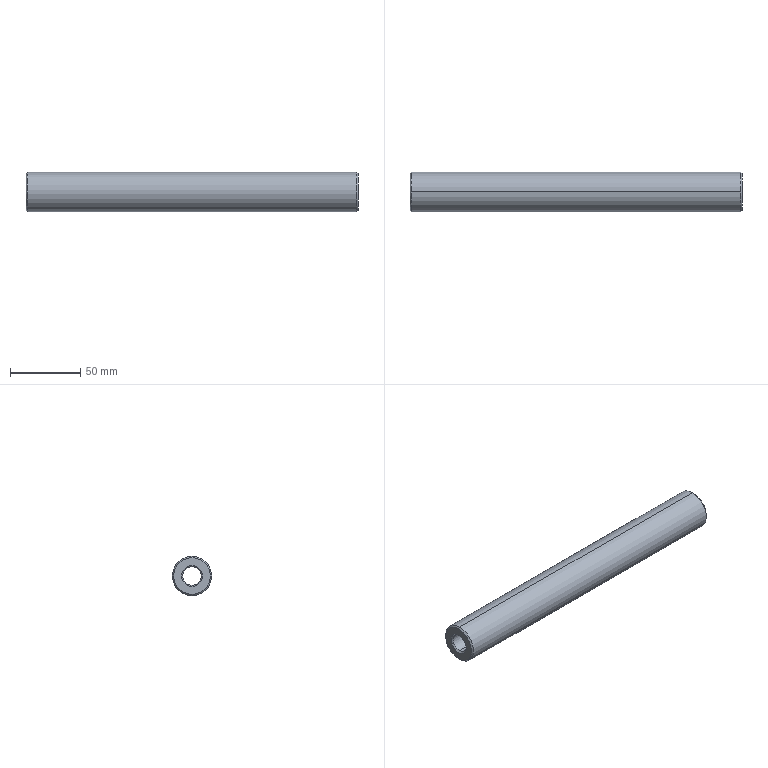Component | SolidWorks | LocatingGuideBushing156-2 | 1 solid | 14 faces | box 236 x 28 x 28 mm | volume 113864 mm3 | cone 8 | cylinder 4 | plane 2 | commonest cylinder face diameters 13 x2 28 x2
build123d program:
from build123d import *

# Parameters (mm, degrees)
SKETCH1_R           = 14
SKETCH1_R_2         = 6.5
BOSS_EXTRUDE1_DEPTH = 236
CHAMFER1_SIZE       = 1


with BuildPart() as part:
    # Sketch1 → Boss-Extrude1 (new body)
    with BuildSketch(Plane.XY):
        Circle(SKETCH1_R)
        Circle(SKETCH1_R_2, mode=Mode.SUBTRACT)
    extrude(amount=BOSS_EXTRUDE1_DEPTH)

    # Chamfer1
    chamfer1_edges = [part.edges().sort_by_distance(p)[0] for p in [
        (-14, 0, 0),
        (-14, 0, 236),
        (-6.5, 0, 0),
        (-6.5, 0, 236),
    ]]
    chamfer(chamfer1_edges, length=CHAMFER1_SIZE)


solid = part.part

# Placed as in the assembly
solid = solid.moved(Location((-455.809, -229.181, 0), (0, 90, 0)))
STEP:
#1=COLOUR_RGB('',0.7922,0.8196,0.9333);
#2=FILL_AREA_STYLE_COLOUR('',#1);
#3=FILL_AREA_STYLE('',(#2));
#4=SURFACE_STYLE_FILL_AREA(#3);
#5=SURFACE_SIDE_STYLE('',(#4));
#6=SURFACE_STYLE_USAGE(.BOTH.,#5);
#7=PRESENTATION_STYLE_ASSIGNMENT((#6));
#8=CARTESIAN_POINT('',(-8.654,-9.023,-0.5118));
#9=VERTEX_POINT('',#8);
#10=CARTESIAN_POINT('',(-8.654,-9.023,0.5118));
#11=VERTEX_POINT('',#10);
#12=CARTESIAN_POINT('',(-8.654,-9.023,-0.));
#13=DIRECTION('',(1.,-0.,0.));
#14=DIRECTION('',(0.,0.,-1.));
#15=AXIS2_PLACEMENT_3D('',#12,#13,#14);
#16=CIRCLE('',#15,0.5118);
#17=EDGE_CURVE('',#9,#11,#16,.T.);
#18=ORIENTED_EDGE('',*,*,#17,.F.);
#19=CARTESIAN_POINT('',(-8.693,-9.023,-0.5512));
#20=VERTEX_POINT('',#19);
#21=CARTESIAN_POINT('',(-8.654,-9.023,-0.5118));
#22=DIRECTION('',(-0.7071,0.,-0.7071));
#23=VECTOR('',#22,39.37);
#24=LINE('',#21,#23);
#25=EDGE_CURVE('',#9,#20,#24,.T.);
#26=ORIENTED_EDGE('',*,*,#25,.T.);
#27=CARTESIAN_POINT('',(-8.693,-9.023,0.5512));
#28=VERTEX_POINT('',#27);
#29=CARTESIAN_POINT('',(-8.693,-9.023,-0.));
#30=DIRECTION('',(-1.,0.,-0.));
#31=DIRECTION('',(0.,0.,-1.));
#32=AXIS2_PLACEMENT_3D('',#29,#30,#31);
#33=CIRCLE('',#32,0.5512);
#34=EDGE_CURVE('',#28,#20,#33,.T.);
#35=ORIENTED_EDGE('',*,*,#34,.F.);
#36=CARTESIAN_POINT('',(-8.654,-9.023,0.5118));
#37=DIRECTION('',(-0.7071,-0.,0.7071));
#38=VECTOR('',#37,39.37);
#39=LINE('',#36,#38);
#40=EDGE_CURVE('',#11,#28,#39,.T.);
#41=ORIENTED_EDGE('',*,*,#40,.F.);
#42=EDGE_LOOP('',(#18,#26,#35,#41));
#43=FACE_OUTER_BOUND('',#42,.T.);
#44=CARTESIAN_POINT('',(-8.654,-9.023,-0.));
#45=DIRECTION('',(-1.,0.,-0.));
#46=DIRECTION('',(0.,0.,1.));
#47=AXIS2_PLACEMENT_3D('',#44,#45,#46);
#48=CONICAL_SURFACE('',#47,0.5118,0.7854);
#49=ADVANCED_FACE('',(#43),#48,.T.);
#50=CARTESIAN_POINT('',(-8.693,-9.023,0.2559));
#51=VERTEX_POINT('',#50);
#52=CARTESIAN_POINT('',(-8.693,-9.023,-0.2559));
#53=VERTEX_POINT('',#52);
#54=CARTESIAN_POINT('',(-8.693,-9.023,-0.));
#55=DIRECTION('',(1.,-0.,0.));
#56=DIRECTION('',(0.,0.,-1.));
#57=AXIS2_PLACEMENT_3D('',#54,#55,#56);
#58=CIRCLE('',#57,0.2559);
#59=EDGE_CURVE('',#51,#53,#58,.T.);
#60=ORIENTED_EDGE('',*,*,#59,.F.);
#61=CARTESIAN_POINT('',(-8.654,-9.023,0.2953));
#62=VERTEX_POINT('',#61);
#63=CARTESIAN_POINT('',(-8.693,-9.023,0.2559));
#64=DIRECTION('',(0.7071,-0.,0.7071));
#65=VECTOR('',#64,39.37);
#66=LINE('',#63,#65);
#67=EDGE_CURVE('',#51,#62,#66,.T.);
#68=ORIENTED_EDGE('',*,*,#67,.T.);
#69=CARTESIAN_POINT('',(-8.654,-9.023,-0.2953));
#70=VERTEX_POINT('',#69);
#71=CARTESIAN_POINT('',(-8.654,-9.023,-0.));
#72=DIRECTION('',(-1.,0.,-0.));
#73=DIRECTION('',(0.,0.,-1.));
#74=AXIS2_PLACEMENT_3D('',#71,#72,#73);
#75=CIRCLE('',#74,0.2953);
#76=EDGE_CURVE('',#70,#62,#75,.T.);
#77=ORIENTED_EDGE('',*,*,#76,.F.);
#78=CARTESIAN_POINT('',(-8.693,-9.023,-0.2559));
#79=DIRECTION('',(0.7071,0.,-0.7071));
#80=VECTOR('',#79,39.37);
#81=LINE('',#78,#80);
#82=EDGE_CURVE('',#53,#70,#81,.T.);
#83=ORIENTED_EDGE('',*,*,#82,.F.);
#84=EDGE_LOOP('',(#60,#68,#77,#83));
#85=FACE_OUTER_BOUND('',#84,.T.);
#86=CARTESIAN_POINT('',(-8.693,-9.023,-0.));
#87=DIRECTION('',(1.,-0.,0.));
#88=DIRECTION('',(0.,0.,-1.));
#89=AXIS2_PLACEMENT_3D('',#86,#87,#88);
#90=CONICAL_SURFACE('',#89,0.2559,0.7854);
#91=ADVANCED_FACE('',(#85),#90,.F.);
#92=CARTESIAN_POINT('',(-17.945,-9.023,0.5118));
#93=VERTEX_POINT('',#92);
#94=CARTESIAN_POINT('',(-17.945,-9.023,-0.5118));
#95=VERTEX_POINT('',#94);
#96=CARTESIAN_POINT('',(-17.945,-9.023,-0.));
#97=DIRECTION('',(-1.,0.,-0.));
#98=DIRECTION('',(0.,0.,-1.));
#99=AXIS2_PLACEMENT_3D('',#96,#97,#98);
#100=CIRCLE('',#99,0.5118);
#101=EDGE_CURVE('',#93,#95,#100,.T.);
#102=ORIENTED_EDGE('',*,*,#101,.F.);
#103=CARTESIAN_POINT('',(-17.906,-9.023,0.5512));
#104=VERTEX_POINT('',#103);
#105=CARTESIAN_POINT('',(-17.906,-9.023,0.5512));
#106=DIRECTION('',(0.7071,-0.,0.7071));
#107=VECTOR('',#106,39.37);
#108=LINE('',#105,#107);
#109=EDGE_CURVE('',#93,#104,#108,.T.);
#110=ORIENTED_EDGE('',*,*,#109,.T.);
#111=CARTESIAN_POINT('',(-17.906,-9.023,-0.5512));
#112=VERTEX_POINT('',#111);
#113=CARTESIAN_POINT('',(-17.906,-9.023,-0.));
#114=DIRECTION('',(1.,-0.,0.));
#115=DIRECTION('',(0.,0.,-1.));
#116=AXIS2_PLACEMENT_3D('',#113,#114,#115);
#117=CIRCLE('',#116,0.5512);
#118=EDGE_CURVE('',#112,#104,#117,.T.);
#119=ORIENTED_EDGE('',*,*,#118,.F.);
#120=CARTESIAN_POINT('',(-17.906,-9.023,-0.5512));
#121=DIRECTION('',(0.7071,0.,-0.7071));
#122=VECTOR('',#121,39.37);
#123=LINE('',#120,#122);
#124=EDGE_CURVE('',#95,#112,#123,.T.);
#125=ORIENTED_EDGE('',*,*,#124,.F.);
#126=EDGE_LOOP('',(#102,#110,#119,#125));
#127=FACE_OUTER_BOUND('',#126,.T.);
#128=CARTESIAN_POINT('',(-17.906,-9.023,-0.));
#129=DIRECTION('',(1.,-0.,0.));
#130=DIRECTION('',(0.,0.,-1.));
#131=AXIS2_PLACEMENT_3D('',#128,#129,#130);
#132=CONICAL_SURFACE('',#131,0.5512,0.7854);
#133=ADVANCED_FACE('',(#127),#132,.T.);
#134=CARTESIAN_POINT('',(-17.906,-9.023,-0.2559));
#135=VERTEX_POINT('',#134);
#136=CARTESIAN_POINT('',(-17.906,-9.023,0.2559));
#137=VERTEX_POINT('',#136);
#138=CARTESIAN_POINT('',(-17.906,-9.023,-0.));
#139=DIRECTION('',(-1.,0.,-0.));
#140=DIRECTION('',(0.,-0.,-1.));
#141=AXIS2_PLACEMENT_3D('',#138,#139,#140);
#142=CIRCLE('',#141,0.2559);
#143=EDGE_CURVE('',#135,#137,#142,.T.);
#144=ORIENTED_EDGE('',*,*,#143,.F.);
#145=CARTESIAN_POINT('',(-17.945,-9.023,-0.2953));
#146=VERTEX_POINT('',#145);
#147=CARTESIAN_POINT('',(-17.945,-9.023,-0.2953));
#148=DIRECTION('',(-0.7071,0.,-0.7071));
#149=VECTOR('',#148,39.37);
#150=LINE('',#147,#149);
#151=EDGE_CURVE('',#135,#146,#150,.T.);
#152=ORIENTED_EDGE('',*,*,#151,.T.);
#153=CARTESIAN_POINT('',(-17.945,-9.023,0.2953));
#154=VERTEX_POINT('',#153);
#155=CARTESIAN_POINT('',(-17.945,-9.023,-0.));
#156=DIRECTION('',(1.,-0.,0.));
#157=DIRECTION('',(0.,0.,-1.));
#158=AXIS2_PLACEMENT_3D('',#155,#156,#157);
#159=CIRCLE('',#158,0.2953);
#160=EDGE_CURVE('',#154,#146,#159,.T.);
#161=ORIENTED_EDGE('',*,*,#160,.F.);
#162=CARTESIAN_POINT('',(-17.945,-9.023,0.2953));
#163=DIRECTION('',(-0.7071,-0.,0.7071));
#164=VECTOR('',#163,39.37);
#165=LINE('',#162,#164);
#166=EDGE_CURVE('',#137,#154,#165,.T.);
#167=ORIENTED_EDGE('',*,*,#166,.F.);
#168=EDGE_LOOP('',(#144,#152,#161,#167));
#169=FACE_OUTER_BOUND('',#168,.T.);
#170=CARTESIAN_POINT('',(-17.945,-9.023,-0.));
#171=DIRECTION('',(-1.,0.,-0.));
#172=DIRECTION('',(0.,0.,1.));
#173=AXIS2_PLACEMENT_3D('',#170,#171,#172);
#174=CONICAL_SURFACE('',#173,0.2953,0.7854);
#175=ADVANCED_FACE('',(#169),#174,.F.);
#176=ORIENTED_EDGE('',*,*,#59,.T.);
#177=CARTESIAN_POINT('',(-8.654,-9.023,-0.2559));
#178=DIRECTION('',(-1.,0.,-0.));
#179=VECTOR('',#178,39.37);
#180=LINE('',#177,#179);
#181=EDGE_CURVE('',#53,#135,#180,.T.);
#182=ORIENTED_EDGE('',*,*,#181,.T.);
#183=ORIENTED_EDGE('',*,*,#143,.T.);
#184=CARTESIAN_POINT('',(-8.654,-9.023,0.2559));
#185=DIRECTION('',(-1.,0.,-0.));
#186=VECTOR('',#185,39.37);
#187=LINE('',#184,#186);
#188=EDGE_CURVE('',#51,#137,#187,.T.);
#189=ORIENTED_EDGE('',*,*,#188,.F.);
#190=EDGE_LOOP('',(#176,#182,#183,#189));
#191=FACE_OUTER_BOUND('',#190,.T.);
#192=CARTESIAN_POINT('',(-8.654,-9.023,-0.));
#193=DIRECTION('',(-1.,0.,-0.));
#194=DIRECTION('',(0.,0.,1.));
#195=AXIS2_PLACEMENT_3D('',#192,#193,#194);
#196=CYLINDRICAL_SURFACE('',#195,0.2559);
#197=ADVANCED_FACE('',(#191),#196,.F.);
#198=ORIENTED_EDGE('',*,*,#34,.T.);
#199=CARTESIAN_POINT('',(-8.654,-9.023,-0.5512));
#200=DIRECTION('',(-1.,0.,-0.));
#201=VECTOR('',#200,39.37);
#202=LINE('',#199,#201);
#203=EDGE_CURVE('',#20,#112,#202,.T.);
#204=ORIENTED_EDGE('',*,*,#203,.T.);
#205=ORIENTED_EDGE('',*,*,#118,.T.);
#206=CARTESIAN_POINT('',(-8.654,-9.023,0.5512));
#207=DIRECTION('',(-1.,0.,-0.));
#208=VECTOR('',#207,39.37);
#209=LINE('',#206,#208);
#210=EDGE_CURVE('',#28,#104,#209,.T.);
#211=ORIENTED_EDGE('',*,*,#210,.F.);
#212=EDGE_LOOP('',(#198,#204,#205,#211));
#213=FACE_OUTER_BOUND('',#212,.T.);
#214=CARTESIAN_POINT('',(-8.654,-9.023,-0.));
#215=DIRECTION('',(-1.,0.,-0.));
#216=DIRECTION('',(0.,0.,1.));
#217=AXIS2_PLACEMENT_3D('',#214,#215,#216);
#218=CYLINDRICAL_SURFACE('',#217,0.5512);
#219=ADVANCED_FACE('',(#213),#218,.T.);
#220=ORIENTED_EDGE('',*,*,#76,.T.);
#221=CARTESIAN_POINT('',(-8.654,-9.023,-0.));
#222=DIRECTION('',(-1.,0.,-0.));
#223=DIRECTION('',(0.,0.,-1.));
#224=AXIS2_PLACEMENT_3D('',#221,#222,#223);
#225=CIRCLE('',#224,0.2953);
#226=EDGE_CURVE('',#62,#70,#225,.T.);
#227=ORIENTED_EDGE('',*,*,#226,.T.);
#228=EDGE_LOOP('',(#220,#227));
#229=FACE_BOUND('',#228,.T.);
#230=CARTESIAN_POINT('',(-8.654,-9.023,-0.));
#231=DIRECTION('',(1.,-0.,0.));
#232=DIRECTION('',(0.,0.,-1.));
#233=AXIS2_PLACEMENT_3D('',#230,#231,#232);
#234=CIRCLE('',#233,0.5118);
#235=EDGE_CURVE('',#11,#9,#234,.T.);
#236=ORIENTED_EDGE('',*,*,#235,.T.);
#237=ORIENTED_EDGE('',*,*,#17,.T.);
#238=EDGE_LOOP('',(#236,#237));
#239=FACE_OUTER_BOUND('',#238,.T.);
#240=CARTESIAN_POINT('',(-8.654,-9.023,-0.));
#241=DIRECTION('',(1.,-0.,0.));
#242=DIRECTION('',(0.,0.,-1.));
#243=AXIS2_PLACEMENT_3D('',#240,#241,#242);
#244=PLANE('',#243);
#245=ADVANCED_FACE('',(#229,#239),#244,.T.);
#246=ORIENTED_EDGE('',*,*,#160,.T.);
#247=CARTESIAN_POINT('',(-17.945,-9.023,-0.));
#248=DIRECTION('',(1.,-0.,0.));
#249=DIRECTION('',(0.,0.,-1.));
#250=AXIS2_PLACEMENT_3D('',#247,#248,#249);
#251=CIRCLE('',#250,0.2953);
#252=EDGE_CURVE('',#146,#154,#251,.T.);
#253=ORIENTED_EDGE('',*,*,#252,.T.);
#254=EDGE_LOOP('',(#246,#253));
#255=FACE_BOUND('',#254,.T.);
#256=CARTESIAN_POINT('',(-17.945,-9.023,-0.));
#257=DIRECTION('',(-1.,0.,-0.));
#258=DIRECTION('',(0.,0.,-1.));
#259=AXIS2_PLACEMENT_3D('',#256,#257,#258);
#260=CIRCLE('',#259,0.5118);
#261=EDGE_CURVE('',#95,#93,#260,.T.);
#262=ORIENTED_EDGE('',*,*,#261,.T.);
#263=ORIENTED_EDGE('',*,*,#101,.T.);
#264=EDGE_LOOP('',(#262,#263));
#265=FACE_OUTER_BOUND('',#264,.T.);
#266=CARTESIAN_POINT('',(-17.945,-9.023,-0.));
#267=DIRECTION('',(1.,-0.,0.));
#268=DIRECTION('',(0.,0.,-1.));
#269=AXIS2_PLACEMENT_3D('',#266,#267,#268);
#270=PLANE('',#269);
#271=ADVANCED_FACE('',(#255,#265),#270,.F.);
#272=ORIENTED_EDGE('',*,*,#203,.F.);
#273=CARTESIAN_POINT('',(-8.693,-9.023,-0.));
#274=DIRECTION('',(-1.,0.,-0.));
#275=DIRECTION('',(0.,0.,-1.));
#276=AXIS2_PLACEMENT_3D('',#273,#274,#275);
#277=CIRCLE('',#276,0.5512);
#278=EDGE_CURVE('',#20,#28,#277,.T.);
#279=ORIENTED_EDGE('',*,*,#278,.T.);
#280=ORIENTED_EDGE('',*,*,#210,.T.);
#281=CARTESIAN_POINT('',(-17.906,-9.023,-0.));
#282=DIRECTION('',(1.,-0.,0.));
#283=DIRECTION('',(0.,0.,-1.));
#284=AXIS2_PLACEMENT_3D('',#281,#282,#283);
#285=CIRCLE('',#284,0.5512);
#286=EDGE_CURVE('',#104,#112,#285,.T.);
#287=ORIENTED_EDGE('',*,*,#286,.T.);
#288=EDGE_LOOP('',(#272,#279,#280,#287));
#289=FACE_OUTER_BOUND('',#288,.T.);
#290=CARTESIAN_POINT('',(-8.654,-9.023,-0.));
#291=DIRECTION('',(-1.,0.,-0.));
#292=DIRECTION('',(0.,0.,1.));
#293=AXIS2_PLACEMENT_3D('',#290,#291,#292);
#294=CYLINDRICAL_SURFACE('',#293,0.5512);
#295=ADVANCED_FACE('',(#289),#294,.T.);
#296=ORIENTED_EDGE('',*,*,#181,.F.);
#297=CARTESIAN_POINT('',(-8.693,-9.023,-0.));
#298=DIRECTION('',(1.,-0.,0.));
#299=DIRECTION('',(0.,0.,-1.));
#300=AXIS2_PLACEMENT_3D('',#297,#298,#299);
#301=CIRCLE('',#300,0.2559);
#302=EDGE_CURVE('',#53,#51,#301,.T.);
#303=ORIENTED_EDGE('',*,*,#302,.T.);
#304=ORIENTED_EDGE('',*,*,#188,.T.);
#305=CARTESIAN_POINT('',(-17.906,-9.023,-0.));
#306=DIRECTION('',(-1.,0.,-0.));
#307=DIRECTION('',(0.,0.,-1.));
#308=AXIS2_PLACEMENT_3D('',#305,#306,#307);
#309=CIRCLE('',#308,0.2559);
#310=EDGE_CURVE('',#137,#135,#309,.T.);
#311=ORIENTED_EDGE('',*,*,#310,.T.);
#312=EDGE_LOOP('',(#296,#303,#304,#311));
#313=FACE_OUTER_BOUND('',#312,.T.);
#314=CARTESIAN_POINT('',(-8.654,-9.023,-0.));
#315=DIRECTION('',(-1.,0.,-0.));
#316=DIRECTION('',(0.,0.,1.));
#317=AXIS2_PLACEMENT_3D('',#314,#315,#316);
#318=CYLINDRICAL_SURFACE('',#317,0.2559);
#319=ADVANCED_FACE('',(#313),#318,.F.);
#320=ORIENTED_EDGE('',*,*,#151,.F.);
#321=ORIENTED_EDGE('',*,*,#310,.F.);
#322=ORIENTED_EDGE('',*,*,#166,.T.);
#323=ORIENTED_EDGE('',*,*,#252,.F.);
#324=EDGE_LOOP('',(#320,#321,#322,#323));
#325=FACE_OUTER_BOUND('',#324,.T.);
#326=CARTESIAN_POINT('',(-17.945,-9.023,-0.));
#327=DIRECTION('',(-1.,0.,-0.));
#328=DIRECTION('',(0.,0.,1.));
#329=AXIS2_PLACEMENT_3D('',#326,#327,#328);
#330=CONICAL_SURFACE('',#329,0.2953,0.7854);
#331=ADVANCED_FACE('',(#325),#330,.F.);
#332=ORIENTED_EDGE('',*,*,#109,.F.);
#333=ORIENTED_EDGE('',*,*,#261,.F.);
#334=ORIENTED_EDGE('',*,*,#124,.T.);
#335=ORIENTED_EDGE('',*,*,#286,.F.);
#336=EDGE_LOOP('',(#332,#333,#334,#335));
#337=FACE_OUTER_BOUND('',#336,.T.);
#338=CARTESIAN_POINT('',(-17.906,-9.023,-0.));
#339=DIRECTION('',(1.,-0.,0.));
#340=DIRECTION('',(0.,0.,-1.));
#341=AXIS2_PLACEMENT_3D('',#338,#339,#340);
#342=CONICAL_SURFACE('',#341,0.5512,0.7854);
#343=ADVANCED_FACE('',(#337),#342,.T.);
#344=ORIENTED_EDGE('',*,*,#67,.F.);
#345=ORIENTED_EDGE('',*,*,#302,.F.);
#346=ORIENTED_EDGE('',*,*,#82,.T.);
#347=ORIENTED_EDGE('',*,*,#226,.F.);
#348=EDGE_LOOP('',(#344,#345,#346,#347));
#349=FACE_OUTER_BOUND('',#348,.T.);
#350=CARTESIAN_POINT('',(-8.693,-9.023,-0.));
#351=DIRECTION('',(1.,-0.,0.));
#352=DIRECTION('',(0.,0.,-1.));
#353=AXIS2_PLACEMENT_3D('',#350,#351,#352);
#354=CONICAL_SURFACE('',#353,0.2559,0.7854);
#355=ADVANCED_FACE('',(#349),#354,.F.);
#356=ORIENTED_EDGE('',*,*,#25,.F.);
#357=ORIENTED_EDGE('',*,*,#235,.F.);
#358=ORIENTED_EDGE('',*,*,#40,.T.);
#359=ORIENTED_EDGE('',*,*,#278,.F.);
#360=EDGE_LOOP('',(#356,#357,#358,#359));
#361=FACE_OUTER_BOUND('',#360,.T.);
#362=CARTESIAN_POINT('',(-8.654,-9.023,-0.));
#363=DIRECTION('',(-1.,0.,-0.));
#364=DIRECTION('',(0.,0.,1.));
#365=AXIS2_PLACEMENT_3D('',#362,#363,#364);
#366=CONICAL_SURFACE('',#365,0.5118,0.7854);
#367=ADVANCED_FACE('',(#361),#366,.T.);
#368=CLOSED_SHELL('',(#49,#91,#133,#175,#197,#219,#245,#271,#295,#319,#331,#343,#355,#367));
#369=MANIFOLD_SOLID_BREP('',#368);
#370=STYLED_ITEM('',(#7),#369);
#371=PRESENTATION_LAYER_ASSIGNMENT('','',(#370));
#372=CARTESIAN_POINT('',(0.,0.,0.));
#373=DIRECTION('',(0.,0.,1.));
#374=DIRECTION('',(1.,0.,0.));
#375=AXIS2_PLACEMENT_3D('',#372,#373,#374);
#376=(LENGTH_UNIT()NAMED_UNIT(*)SI_UNIT($,.METRE.));
#377=LENGTH_MEASURE_WITH_UNIT(LENGTH_MEASURE(0.0254),#376);
#378=DIMENSIONAL_EXPONENTS(1.,0.,0.,0.,0.,0.,0.);
#379=(CONVERSION_BASED_UNIT('',#377)LENGTH_UNIT()NAMED_UNIT(#378));
#380=UNCERTAINTY_MEASURE_WITH_UNIT(LENGTH_MEASURE(0.00001),#379,'','');
#381=(NAMED_UNIT(*)PLANE_ANGLE_UNIT()SI_UNIT($,.RADIAN.));
#382=(NAMED_UNIT(*)SI_UNIT($,.STERADIAN.)SOLID_ANGLE_UNIT());
#383=(GEOMETRIC_REPRESENTATION_CONTEXT(3)GLOBAL_UNCERTAINTY_ASSIGNED_CONTEXT((#380))GLOBAL_UNIT_ASSIGNED_CONTEXT((#379,#381,#382))REPRESENTATION_CONTEXT('',''));
#384=ADVANCED_BREP_SHAPE_REPRESENTATION('',(#369,#375),#383);
#385=(LENGTH_UNIT()NAMED_UNIT(*)SI_UNIT($,.METRE.));
#386=LENGTH_MEASURE_WITH_UNIT(LENGTH_MEASURE(0.0254),#385);
#387=DIMENSIONAL_EXPONENTS(1.,0.,0.,0.,0.,0.,0.);
#388=(CONVERSION_BASED_UNIT('',#386)LENGTH_UNIT()NAMED_UNIT(#387));
#389=UNCERTAINTY_MEASURE_WITH_UNIT(LENGTH_MEASURE(0.00001),#388,'','');
#390=(NAMED_UNIT(*)PLANE_ANGLE_UNIT()SI_UNIT($,.RADIAN.));
#391=(NAMED_UNIT(*)SI_UNIT($,.STERADIAN.)SOLID_ANGLE_UNIT());
#392=(GEOMETRIC_REPRESENTATION_CONTEXT(3)GLOBAL_UNCERTAINTY_ASSIGNED_CONTEXT((#389))GLOBAL_UNIT_ASSIGNED_CONTEXT((#388,#390,#391))REPRESENTATION_CONTEXT('',''));
#393=MECHANICAL_DESIGN_GEOMETRIC_PRESENTATION_REPRESENTATION('',(#370),#392);